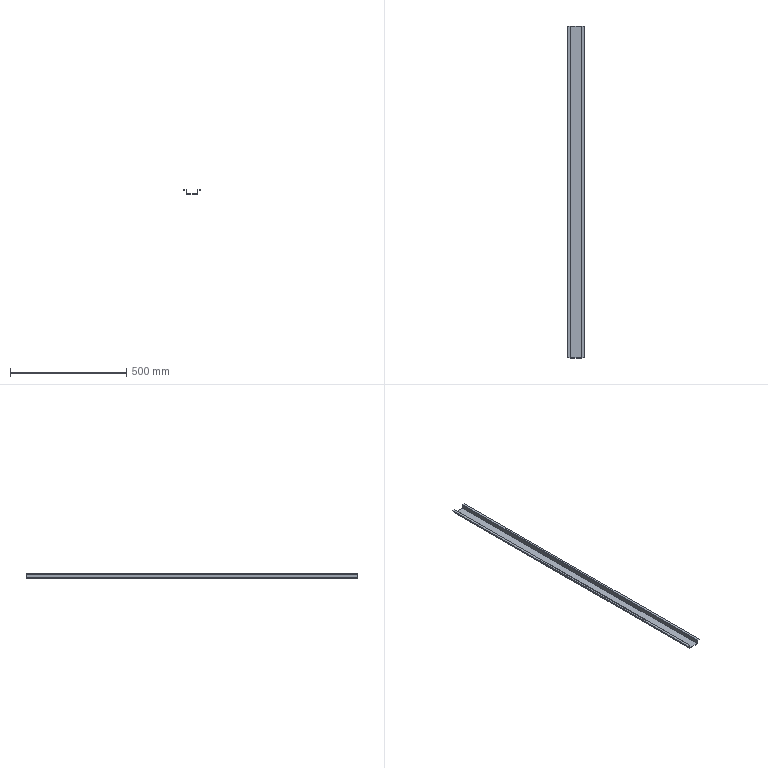Component | SolidWorks | AirFurnaceElectricalCabinet-ElectricalPanelAssembly-1_ElectricalPanelReinforcementPlate-L1425-1 | 1 solid | 38 faces | box 71.6 x 1425 x 18 mm | volume 175929 mm3 | plane 30 | cylinder 8 | commonest cylinder face diameters 3.9 x4 1.5 x4
STEP:
#1=CARTESIAN_POINT('',(8.781,4.854,-4.843));
#2=VERTEX_POINT('',#1);
#3=CARTESIAN_POINT('',(6.967,4.854,-4.843));
#4=VERTEX_POINT('',#3);
#5=CARTESIAN_POINT('',(8.858,4.854,-4.843));
#6=DIRECTION('',(-1.,0.,0.));
#7=VECTOR('',#6,39.37);
#8=LINE('',#5,#7);
#9=EDGE_CURVE('',#2,#4,#8,.T.);
#10=ORIENTED_EDGE('',*,*,#9,.F.);
#11=CARTESIAN_POINT('',(8.781,4.854,-4.795));
#12=VERTEX_POINT('',#11);
#13=CARTESIAN_POINT('',(8.781,4.854,-4.843));
#14=DIRECTION('',(0.,0.,1.));
#15=VECTOR('',#14,39.37);
#16=LINE('',#13,#15);
#17=EDGE_CURVE('',#2,#12,#16,.T.);
#18=ORIENTED_EDGE('',*,*,#17,.T.);
#19=CARTESIAN_POINT('',(6.967,4.854,-4.795));
#20=VERTEX_POINT('',#19);
#21=CARTESIAN_POINT('',(8.858,4.854,-4.795));
#22=DIRECTION('',(-1.,0.,0.));
#23=VECTOR('',#22,39.37);
#24=LINE('',#21,#23);
#25=EDGE_CURVE('',#12,#20,#24,.T.);
#26=ORIENTED_EDGE('',*,*,#25,.T.);
#27=CARTESIAN_POINT('',(6.967,4.854,-4.795));
#28=DIRECTION('',(-0.,0.,-1.));
#29=VECTOR('',#28,39.37);
#30=LINE('',#27,#29);
#31=EDGE_CURVE('',#20,#4,#30,.T.);
#32=ORIENTED_EDGE('',*,*,#31,.T.);
#33=EDGE_LOOP('',(#10,#18,#26,#32));
#34=FACE_OUTER_BOUND('',#33,.T.);
#35=CARTESIAN_POINT('',(8.811,4.854,-4.766));
#36=DIRECTION('',(0.,-1.,0.));
#37=DIRECTION('',(-1.,0.,0.));
#38=AXIS2_PLACEMENT_3D('',#35,#36,#37);
#39=PLANE('',#38);
#40=ADVANCED_FACE('',(#34),#39,.T.);
#41=CARTESIAN_POINT('',(8.781,60.957,-4.843));
#42=VERTEX_POINT('',#41);
#43=CARTESIAN_POINT('',(6.967,60.957,-4.843));
#44=VERTEX_POINT('',#43);
#45=CARTESIAN_POINT('',(8.858,60.957,-4.843));
#46=DIRECTION('',(-1.,0.,0.));
#47=VECTOR('',#46,39.37);
#48=LINE('',#45,#47);
#49=EDGE_CURVE('',#42,#44,#48,.T.);
#50=ORIENTED_EDGE('',*,*,#49,.T.);
#51=CARTESIAN_POINT('',(6.967,60.957,-4.795));
#52=VERTEX_POINT('',#51);
#53=CARTESIAN_POINT('',(6.967,60.957,-4.843));
#54=DIRECTION('',(0.,0.,1.));
#55=VECTOR('',#54,39.37);
#56=LINE('',#53,#55);
#57=EDGE_CURVE('',#44,#52,#56,.T.);
#58=ORIENTED_EDGE('',*,*,#57,.T.);
#59=CARTESIAN_POINT('',(8.781,60.957,-4.795));
#60=VERTEX_POINT('',#59);
#61=CARTESIAN_POINT('',(8.858,60.957,-4.795));
#62=DIRECTION('',(-1.,0.,0.));
#63=VECTOR('',#62,39.37);
#64=LINE('',#61,#63);
#65=EDGE_CURVE('',#60,#52,#64,.T.);
#66=ORIENTED_EDGE('',*,*,#65,.F.);
#67=CARTESIAN_POINT('',(8.781,60.957,-4.795));
#68=DIRECTION('',(-0.,0.,-1.));
#69=VECTOR('',#68,39.37);
#70=LINE('',#67,#69);
#71=EDGE_CURVE('',#60,#42,#70,.T.);
#72=ORIENTED_EDGE('',*,*,#71,.T.);
#73=EDGE_LOOP('',(#50,#58,#66,#72));
#74=FACE_OUTER_BOUND('',#73,.T.);
#75=CARTESIAN_POINT('',(6.937,60.957,-4.766));
#76=DIRECTION('',(0.,1.,0.));
#77=DIRECTION('',(1.,0.,-0.));
#78=AXIS2_PLACEMENT_3D('',#75,#76,#77);
#79=PLANE('',#78);
#80=ADVANCED_FACE('',(#74),#79,.T.);
#81=ORIENTED_EDGE('',*,*,#49,.F.);
#82=CARTESIAN_POINT('',(8.781,4.854,-4.843));
#83=DIRECTION('',(0.,1.,0.));
#84=VECTOR('',#83,39.37);
#85=LINE('',#82,#84);
#86=EDGE_CURVE('',#2,#42,#85,.T.);
#87=ORIENTED_EDGE('',*,*,#86,.F.);
#88=ORIENTED_EDGE('',*,*,#9,.T.);
#89=CARTESIAN_POINT('',(6.967,4.854,-4.843));
#90=DIRECTION('',(0.,1.,0.));
#91=VECTOR('',#90,39.37);
#92=LINE('',#89,#91);
#93=EDGE_CURVE('',#4,#44,#92,.T.);
#94=ORIENTED_EDGE('',*,*,#93,.T.);
#95=EDGE_LOOP('',(#81,#87,#88,#94));
#96=FACE_OUTER_BOUND('',#95,.T.);
#97=CARTESIAN_POINT('',(8.858,4.854,-4.843));
#98=DIRECTION('',(-0.,0.,-1.));
#99=DIRECTION('',(1.,0.,-0.));
#100=AXIS2_PLACEMENT_3D('',#97,#98,#99);
#101=PLANE('',#100);
#102=ADVANCED_FACE('',(#96),#101,.T.);
#103=ORIENTED_EDGE('',*,*,#65,.T.);
#104=CARTESIAN_POINT('',(6.967,4.854,-4.795));
#105=DIRECTION('',(0.,1.,0.));
#106=VECTOR('',#105,39.37);
#107=LINE('',#104,#106);
#108=EDGE_CURVE('',#20,#52,#107,.T.);
#109=ORIENTED_EDGE('',*,*,#108,.F.);
#110=ORIENTED_EDGE('',*,*,#25,.F.);
#111=CARTESIAN_POINT('',(8.781,4.854,-4.795));
#112=DIRECTION('',(0.,1.,0.));
#113=VECTOR('',#112,39.37);
#114=LINE('',#111,#113);
#115=EDGE_CURVE('',#12,#60,#114,.T.);
#116=ORIENTED_EDGE('',*,*,#115,.T.);
#117=EDGE_LOOP('',(#103,#109,#110,#116));
#118=FACE_OUTER_BOUND('',#117,.T.);
#119=CARTESIAN_POINT('',(8.858,4.854,-4.795));
#120=DIRECTION('',(-0.,0.,-1.));
#121=DIRECTION('',(1.,0.,-0.));
#122=AXIS2_PLACEMENT_3D('',#119,#120,#121);
#123=PLANE('',#122);
#124=ADVANCED_FACE('',(#118),#123,.F.);
#125=ORIENTED_EDGE('',*,*,#31,.F.);
#126=CARTESIAN_POINT('',(6.937,4.854,-4.766));
#127=VERTEX_POINT('',#126);
#128=CARTESIAN_POINT('',(6.967,4.854,-4.766));
#129=DIRECTION('',(0.,1.,0.));
#130=DIRECTION('',(1.,0.,0.));
#131=AXIS2_PLACEMENT_3D('',#128,#129,#130);
#132=CIRCLE('',#131,0.02953);
#133=EDGE_CURVE('',#20,#127,#132,.T.);
#134=ORIENTED_EDGE('',*,*,#133,.T.);
#135=CARTESIAN_POINT('',(6.89,4.854,-4.766));
#136=VERTEX_POINT('',#135);
#137=CARTESIAN_POINT('',(6.89,4.854,-4.766));
#138=DIRECTION('',(1.,0.,-0.));
#139=VECTOR('',#138,39.37);
#140=LINE('',#137,#139);
#141=EDGE_CURVE('',#136,#127,#140,.T.);
#142=ORIENTED_EDGE('',*,*,#141,.F.);
#143=CARTESIAN_POINT('',(6.967,4.854,-4.766));
#144=DIRECTION('',(0.,1.,0.));
#145=DIRECTION('',(1.,0.,0.));
#146=AXIS2_PLACEMENT_3D('',#143,#144,#145);
#147=CIRCLE('',#146,0.07677);
#148=EDGE_CURVE('',#4,#136,#147,.T.);
#149=ORIENTED_EDGE('',*,*,#148,.F.);
#150=EDGE_LOOP('',(#125,#134,#142,#149));
#151=FACE_OUTER_BOUND('',#150,.T.);
#152=CARTESIAN_POINT('',(6.967,4.854,-4.766));
#153=DIRECTION('',(0.,-1.,0.));
#154=DIRECTION('',(-1.,0.,0.));
#155=AXIS2_PLACEMENT_3D('',#152,#153,#154);
#156=PLANE('',#155);
#157=ADVANCED_FACE('',(#151),#156,.T.);
#158=CARTESIAN_POINT('',(6.937,60.957,-4.766));
#159=VERTEX_POINT('',#158);
#160=CARTESIAN_POINT('',(6.89,60.957,-4.766));
#161=VERTEX_POINT('',#160);
#162=CARTESIAN_POINT('',(6.937,60.957,-4.766));
#163=DIRECTION('',(-1.,0.,0.));
#164=VECTOR('',#163,39.37);
#165=LINE('',#162,#164);
#166=EDGE_CURVE('',#159,#161,#165,.T.);
#167=ORIENTED_EDGE('',*,*,#166,.F.);
#168=CARTESIAN_POINT('',(6.967,60.957,-4.766));
#169=DIRECTION('',(0.,-1.,0.));
#170=DIRECTION('',(1.,0.,0.));
#171=AXIS2_PLACEMENT_3D('',#168,#169,#170);
#172=CIRCLE('',#171,0.02953);
#173=EDGE_CURVE('',#159,#52,#172,.T.);
#174=ORIENTED_EDGE('',*,*,#173,.T.);
#175=ORIENTED_EDGE('',*,*,#57,.F.);
#176=CARTESIAN_POINT('',(6.967,60.957,-4.766));
#177=DIRECTION('',(0.,-1.,0.));
#178=DIRECTION('',(-1.,0.,0.));
#179=AXIS2_PLACEMENT_3D('',#176,#177,#178);
#180=CIRCLE('',#179,0.07677);
#181=EDGE_CURVE('',#161,#44,#180,.T.);
#182=ORIENTED_EDGE('',*,*,#181,.F.);
#183=EDGE_LOOP('',(#167,#174,#175,#182));
#184=FACE_OUTER_BOUND('',#183,.T.);
#185=CARTESIAN_POINT('',(6.967,60.957,-4.766));
#186=DIRECTION('',(0.,1.,0.));
#187=DIRECTION('',(1.,0.,-0.));
#188=AXIS2_PLACEMENT_3D('',#185,#186,#187);
#189=PLANE('',#188);
#190=ADVANCED_FACE('',(#184),#189,.T.);
#191=ORIENTED_EDGE('',*,*,#181,.T.);
#192=ORIENTED_EDGE('',*,*,#93,.F.);
#193=ORIENTED_EDGE('',*,*,#148,.T.);
#194=CARTESIAN_POINT('',(6.89,4.854,-4.766));
#195=DIRECTION('',(0.,1.,0.));
#196=VECTOR('',#195,39.37);
#197=LINE('',#194,#196);
#198=EDGE_CURVE('',#136,#161,#197,.T.);
#199=ORIENTED_EDGE('',*,*,#198,.T.);
#200=EDGE_LOOP('',(#191,#192,#193,#199));
#201=FACE_OUTER_BOUND('',#200,.T.);
#202=CARTESIAN_POINT('',(6.967,-23.197,-4.766));
#203=DIRECTION('',(0.,1.,0.));
#204=DIRECTION('',(1.,0.,0.));
#205=AXIS2_PLACEMENT_3D('',#202,#203,#204);
#206=CYLINDRICAL_SURFACE('',#205,0.07677);
#207=ADVANCED_FACE('',(#201),#206,.T.);
#208=ORIENTED_EDGE('',*,*,#173,.F.);
#209=CARTESIAN_POINT('',(6.937,4.854,-4.766));
#210=DIRECTION('',(0.,1.,0.));
#211=VECTOR('',#210,39.37);
#212=LINE('',#209,#211);
#213=EDGE_CURVE('',#127,#159,#212,.T.);
#214=ORIENTED_EDGE('',*,*,#213,.F.);
#215=ORIENTED_EDGE('',*,*,#133,.F.);
#216=ORIENTED_EDGE('',*,*,#108,.T.);
#217=EDGE_LOOP('',(#208,#214,#215,#216));
#218=FACE_OUTER_BOUND('',#217,.T.);
#219=CARTESIAN_POINT('',(6.967,-23.197,-4.766));
#220=DIRECTION('',(0.,1.,0.));
#221=DIRECTION('',(1.,0.,0.));
#222=AXIS2_PLACEMENT_3D('',#219,#220,#221);
#223=CYLINDRICAL_SURFACE('',#222,0.02953);
#224=ADVANCED_FACE('',(#218),#223,.F.);
#225=CARTESIAN_POINT('',(6.465,60.957,-4.181));
#226=VERTEX_POINT('',#225);
#227=CARTESIAN_POINT('',(6.465,60.957,-4.134));
#228=VERTEX_POINT('',#227);
#229=CARTESIAN_POINT('',(6.465,60.957,-4.181));
#230=DIRECTION('',(0.,0.,1.));
#231=VECTOR('',#230,39.37);
#232=LINE('',#229,#231);
#233=EDGE_CURVE('',#226,#228,#232,.T.);
#234=ORIENTED_EDGE('',*,*,#233,.F.);
#235=CARTESIAN_POINT('',(6.465,4.854,-4.181));
#236=VERTEX_POINT('',#235);
#237=CARTESIAN_POINT('',(6.465,4.854,-4.181));
#238=DIRECTION('',(0.,1.,0.));
#239=VECTOR('',#238,39.37);
#240=LINE('',#237,#239);
#241=EDGE_CURVE('',#236,#226,#240,.T.);
#242=ORIENTED_EDGE('',*,*,#241,.F.);
#243=CARTESIAN_POINT('',(6.465,4.854,-4.134));
#244=VERTEX_POINT('',#243);
#245=CARTESIAN_POINT('',(6.465,4.854,-4.181));
#246=DIRECTION('',(0.,0.,1.));
#247=VECTOR('',#246,39.37);
#248=LINE('',#245,#247);
#249=EDGE_CURVE('',#236,#244,#248,.T.);
#250=ORIENTED_EDGE('',*,*,#249,.T.);
#251=CARTESIAN_POINT('',(6.465,4.854,-4.134));
#252=DIRECTION('',(0.,1.,0.));
#253=VECTOR('',#252,39.37);
#254=LINE('',#251,#253);
#255=EDGE_CURVE('',#244,#228,#254,.T.);
#256=ORIENTED_EDGE('',*,*,#255,.T.);
#257=EDGE_LOOP('',(#234,#242,#250,#256));
#258=FACE_OUTER_BOUND('',#257,.T.);
#259=CARTESIAN_POINT('',(6.465,4.854,-4.181));
#260=DIRECTION('',(-1.,0.,0.));
#261=DIRECTION('',(0.,1.,0.));
#262=AXIS2_PLACEMENT_3D('',#259,#260,#261);
#263=PLANE('',#262);
#264=ADVANCED_FACE('',(#258),#263,.T.);
#265=CARTESIAN_POINT('',(6.86,60.957,-4.134));
#266=VERTEX_POINT('',#265);
#267=CARTESIAN_POINT('',(6.89,60.957,-4.134));
#268=DIRECTION('',(-1.,0.,0.));
#269=VECTOR('',#268,39.37);
#270=LINE('',#267,#269);
#271=EDGE_CURVE('',#266,#228,#270,.T.);
#272=ORIENTED_EDGE('',*,*,#271,.F.);
#273=CARTESIAN_POINT('',(6.86,60.957,-4.181));
#274=VERTEX_POINT('',#273);
#275=CARTESIAN_POINT('',(6.86,60.957,-4.134));
#276=DIRECTION('',(-0.,0.,-1.));
#277=VECTOR('',#276,39.37);
#278=LINE('',#275,#277);
#279=EDGE_CURVE('',#266,#274,#278,.T.);
#280=ORIENTED_EDGE('',*,*,#279,.T.);
#281=CARTESIAN_POINT('',(6.89,60.957,-4.181));
#282=DIRECTION('',(-1.,0.,0.));
#283=VECTOR('',#282,39.37);
#284=LINE('',#281,#283);
#285=EDGE_CURVE('',#274,#226,#284,.T.);
#286=ORIENTED_EDGE('',*,*,#285,.T.);
#287=ORIENTED_EDGE('',*,*,#233,.T.);
#288=EDGE_LOOP('',(#272,#280,#286,#287));
#289=FACE_OUTER_BOUND('',#288,.T.);
#290=CARTESIAN_POINT('',(6.86,60.957,-4.211));
#291=DIRECTION('',(0.,1.,0.));
#292=DIRECTION('',(1.,0.,-0.));
#293=AXIS2_PLACEMENT_3D('',#290,#291,#292);
#294=PLANE('',#293);
#295=ADVANCED_FACE('',(#289),#294,.T.);
#296=ORIENTED_EDGE('',*,*,#271,.T.);
#297=ORIENTED_EDGE('',*,*,#255,.F.);
#298=CARTESIAN_POINT('',(6.86,4.854,-4.134));
#299=VERTEX_POINT('',#298);
#300=CARTESIAN_POINT('',(6.89,4.854,-4.134));
#301=DIRECTION('',(-1.,0.,0.));
#302=VECTOR('',#301,39.37);
#303=LINE('',#300,#302);
#304=EDGE_CURVE('',#299,#244,#303,.T.);
#305=ORIENTED_EDGE('',*,*,#304,.F.);
#306=CARTESIAN_POINT('',(6.86,4.854,-4.134));
#307=DIRECTION('',(0.,1.,0.));
#308=VECTOR('',#307,39.37);
#309=LINE('',#306,#308);
#310=EDGE_CURVE('',#299,#266,#309,.T.);
#311=ORIENTED_EDGE('',*,*,#310,.T.);
#312=EDGE_LOOP('',(#296,#297,#305,#311));
#313=FACE_OUTER_BOUND('',#312,.T.);
#314=CARTESIAN_POINT('',(6.89,4.854,-4.134));
#315=DIRECTION('',(0.,0.,-1.));
#316=DIRECTION('',(1.,0.,0.));
#317=AXIS2_PLACEMENT_3D('',#314,#315,#316);
#318=PLANE('',#317);
#319=ADVANCED_FACE('',(#313),#318,.F.);
#320=CARTESIAN_POINT('',(6.86,4.854,-4.181));
#321=VERTEX_POINT('',#320);
#322=CARTESIAN_POINT('',(6.89,4.854,-4.181));
#323=DIRECTION('',(-1.,0.,0.));
#324=VECTOR('',#323,39.37);
#325=LINE('',#322,#324);
#326=EDGE_CURVE('',#321,#236,#325,.T.);
#327=ORIENTED_EDGE('',*,*,#326,.F.);
#328=CARTESIAN_POINT('',(6.86,4.854,-4.181));
#329=DIRECTION('',(0.,0.,1.));
#330=VECTOR('',#329,39.37);
#331=LINE('',#328,#330);
#332=EDGE_CURVE('',#321,#299,#331,.T.);
#333=ORIENTED_EDGE('',*,*,#332,.T.);
#334=ORIENTED_EDGE('',*,*,#304,.T.);
#335=ORIENTED_EDGE('',*,*,#249,.F.);
#336=EDGE_LOOP('',(#327,#333,#334,#335));
#337=FACE_OUTER_BOUND('',#336,.T.);
#338=CARTESIAN_POINT('',(6.937,4.854,-4.211));
#339=DIRECTION('',(0.,-1.,0.));
#340=DIRECTION('',(-1.,0.,0.));
#341=AXIS2_PLACEMENT_3D('',#338,#339,#340);
#342=PLANE('',#341);
#343=ADVANCED_FACE('',(#337),#342,.T.);
#344=ORIENTED_EDGE('',*,*,#285,.F.);
#345=CARTESIAN_POINT('',(6.86,4.854,-4.181));
#346=DIRECTION('',(0.,1.,0.));
#347=VECTOR('',#346,39.37);
#348=LINE('',#345,#347);
#349=EDGE_CURVE('',#321,#274,#348,.T.);
#350=ORIENTED_EDGE('',*,*,#349,.F.);
#351=ORIENTED_EDGE('',*,*,#326,.T.);
#352=ORIENTED_EDGE('',*,*,#241,.T.);
#353=EDGE_LOOP('',(#344,#350,#351,#352));
#354=FACE_OUTER_BOUND('',#353,.T.);
#355=CARTESIAN_POINT('',(6.89,4.854,-4.181));
#356=DIRECTION('',(0.,0.,-1.));
#357=DIRECTION('',(1.,0.,0.));
#358=AXIS2_PLACEMENT_3D('',#355,#356,#357);
#359=PLANE('',#358);
#360=ADVANCED_FACE('',(#354),#359,.T.);
#361=ORIENTED_EDGE('',*,*,#279,.F.);
#362=CARTESIAN_POINT('',(6.937,60.957,-4.211));
#363=VERTEX_POINT('',#362);
#364=CARTESIAN_POINT('',(6.86,60.957,-4.211));
#365=DIRECTION('',(0.,1.,0.));
#366=DIRECTION('',(0.,0.,-1.));
#367=AXIS2_PLACEMENT_3D('',#364,#365,#366);
#368=CIRCLE('',#367,0.07677);
#369=EDGE_CURVE('',#266,#363,#368,.T.);
#370=ORIENTED_EDGE('',*,*,#369,.T.);
#371=CARTESIAN_POINT('',(6.89,60.957,-4.211));
#372=VERTEX_POINT('',#371);
#373=CARTESIAN_POINT('',(6.89,60.957,-4.211));
#374=DIRECTION('',(1.,0.,-0.));
#375=VECTOR('',#374,39.37);
#376=LINE('',#373,#375);
#377=EDGE_CURVE('',#372,#363,#376,.T.);
#378=ORIENTED_EDGE('',*,*,#377,.F.);
#379=CARTESIAN_POINT('',(6.86,60.957,-4.211));
#380=DIRECTION('',(0.,1.,0.));
#381=DIRECTION('',(0.,0.,-1.));
#382=AXIS2_PLACEMENT_3D('',#379,#380,#381);
#383=CIRCLE('',#382,0.02953);
#384=EDGE_CURVE('',#274,#372,#383,.T.);
#385=ORIENTED_EDGE('',*,*,#384,.F.);
#386=EDGE_LOOP('',(#361,#370,#378,#385));
#387=FACE_OUTER_BOUND('',#386,.T.);
#388=CARTESIAN_POINT('',(6.86,60.957,-4.211));
#389=DIRECTION('',(0.,-1.,0.));
#390=DIRECTION('',(-0.,0.,1.));
#391=AXIS2_PLACEMENT_3D('',#388,#389,#390);
#392=PLANE('',#391);
#393=ADVANCED_FACE('',(#387),#392,.F.);
#394=ORIENTED_EDGE('',*,*,#369,.F.);
#395=ORIENTED_EDGE('',*,*,#310,.F.);
#396=CARTESIAN_POINT('',(6.937,4.854,-4.211));
#397=VERTEX_POINT('',#396);
#398=CARTESIAN_POINT('',(6.86,4.854,-4.211));
#399=DIRECTION('',(0.,-1.,0.));
#400=DIRECTION('',(0.,0.,-1.));
#401=AXIS2_PLACEMENT_3D('',#398,#399,#400);
#402=CIRCLE('',#401,0.07677);
#403=EDGE_CURVE('',#397,#299,#402,.T.);
#404=ORIENTED_EDGE('',*,*,#403,.F.);
#405=CARTESIAN_POINT('',(6.937,4.854,-4.211));
#406=DIRECTION('',(0.,1.,0.));
#407=VECTOR('',#406,39.37);
#408=LINE('',#405,#407);
#409=EDGE_CURVE('',#397,#363,#408,.T.);
#410=ORIENTED_EDGE('',*,*,#409,.T.);
#411=EDGE_LOOP('',(#394,#395,#404,#410));
#412=FACE_OUTER_BOUND('',#411,.T.);
#413=CARTESIAN_POINT('',(6.86,-23.197,-4.211));
#414=DIRECTION('',(0.,1.,0.));
#415=DIRECTION('',(0.,0.,-1.));
#416=AXIS2_PLACEMENT_3D('',#413,#414,#415);
#417=CYLINDRICAL_SURFACE('',#416,0.07677);
#418=ADVANCED_FACE('',(#412),#417,.T.);
#419=CARTESIAN_POINT('',(6.89,4.854,-4.211));
#420=VERTEX_POINT('',#419);
#421=CARTESIAN_POINT('',(6.937,4.854,-4.211));
#422=DIRECTION('',(-1.,0.,0.));
#423=VECTOR('',#422,39.37);
#424=LINE('',#421,#423);
#425=EDGE_CURVE('',#397,#420,#424,.T.);
#426=ORIENTED_EDGE('',*,*,#425,.F.);
#427=ORIENTED_EDGE('',*,*,#403,.T.);
#428=ORIENTED_EDGE('',*,*,#332,.F.);
#429=CARTESIAN_POINT('',(6.86,4.854,-4.211));
#430=DIRECTION('',(0.,-1.,0.));
#431=DIRECTION('',(0.,0.,1.));
#432=AXIS2_PLACEMENT_3D('',#429,#430,#431);
#433=CIRCLE('',#432,0.02953);
#434=EDGE_CURVE('',#420,#321,#433,.T.);
#435=ORIENTED_EDGE('',*,*,#434,.F.);
#436=EDGE_LOOP('',(#426,#427,#428,#435));
#437=FACE_OUTER_BOUND('',#436,.T.);
#438=CARTESIAN_POINT('',(6.86,4.854,-4.211));
#439=DIRECTION('',(0.,1.,0.));
#440=DIRECTION('',(0.,0.,-1.));
#441=AXIS2_PLACEMENT_3D('',#438,#439,#440);
#442=PLANE('',#441);
#443=ADVANCED_FACE('',(#437),#442,.F.);
#444=ORIENTED_EDGE('',*,*,#384,.T.);
#445=CARTESIAN_POINT('',(6.89,4.854,-4.211));
#446=DIRECTION('',(0.,1.,0.));
#447=VECTOR('',#446,39.37);
#448=LINE('',#445,#447);
#449=EDGE_CURVE('',#420,#372,#448,.T.);
#450=ORIENTED_EDGE('',*,*,#449,.F.);
#451=ORIENTED_EDGE('',*,*,#434,.T.);
#452=ORIENTED_EDGE('',*,*,#349,.T.);
#453=EDGE_LOOP('',(#444,#450,#451,#452));
#454=FACE_OUTER_BOUND('',#453,.T.);
#455=CARTESIAN_POINT('',(6.86,-23.197,-4.211));
#456=DIRECTION('',(0.,1.,0.));
#457=DIRECTION('',(0.,0.,-1.));
#458=AXIS2_PLACEMENT_3D('',#455,#456,#457);
#459=CYLINDRICAL_SURFACE('',#458,0.02953);
#460=ADVANCED_FACE('',(#454),#459,.F.);
#461=CARTESIAN_POINT('',(6.89,60.957,-4.843));
#462=DIRECTION('',(0.,0.,1.));
#463=VECTOR('',#462,39.37);
#464=LINE('',#461,#463);
#465=EDGE_CURVE('',#161,#372,#464,.T.);
#466=ORIENTED_EDGE('',*,*,#465,.F.);
#467=ORIENTED_EDGE('',*,*,#198,.F.);
#468=CARTESIAN_POINT('',(6.89,4.854,-4.843));
#469=DIRECTION('',(0.,0.,1.));
#470=VECTOR('',#469,39.37);
#471=LINE('',#468,#470);
#472=EDGE_CURVE('',#136,#420,#471,.T.);
#473=ORIENTED_EDGE('',*,*,#472,.T.);
#474=ORIENTED_EDGE('',*,*,#449,.T.);
#475=EDGE_LOOP('',(#466,#467,#473,#474));
#476=FACE_OUTER_BOUND('',#475,.T.);
#477=CARTESIAN_POINT('',(6.89,4.854,-4.843));
#478=DIRECTION('',(-1.,0.,0.));
#479=DIRECTION('',(0.,1.,0.));
#480=AXIS2_PLACEMENT_3D('',#477,#478,#479);
#481=PLANE('',#480);
#482=ADVANCED_FACE('',(#476),#481,.T.);
#483=ORIENTED_EDGE('',*,*,#472,.F.);
#484=ORIENTED_EDGE('',*,*,#141,.T.);
#485=CARTESIAN_POINT('',(6.937,4.854,-4.843));
#486=DIRECTION('',(0.,0.,1.));
#487=VECTOR('',#486,39.37);
#488=LINE('',#485,#487);
#489=EDGE_CURVE('',#127,#397,#488,.T.);
#490=ORIENTED_EDGE('',*,*,#489,.T.);
#491=ORIENTED_EDGE('',*,*,#425,.T.);
#492=EDGE_LOOP('',(#483,#484,#490,#491));
#493=FACE_OUTER_BOUND('',#492,.T.);
#494=CARTESIAN_POINT('',(6.967,4.854,-4.795));
#495=DIRECTION('',(0.,-1.,0.));
#496=DIRECTION('',(-1.,0.,0.));
#497=AXIS2_PLACEMENT_3D('',#494,#495,#496);
#498=PLANE('',#497);
#499=ADVANCED_FACE('',(#493),#498,.T.);
#500=CARTESIAN_POINT('',(6.937,60.957,-4.843));
#501=DIRECTION('',(0.,0.,1.));
#502=VECTOR('',#501,39.37);
#503=LINE('',#500,#502);
#504=EDGE_CURVE('',#159,#363,#503,.T.);
#505=ORIENTED_EDGE('',*,*,#504,.T.);
#506=ORIENTED_EDGE('',*,*,#409,.F.);
#507=ORIENTED_EDGE('',*,*,#489,.F.);
#508=ORIENTED_EDGE('',*,*,#213,.T.);
#509=EDGE_LOOP('',(#505,#506,#507,#508));
#510=FACE_OUTER_BOUND('',#509,.T.);
#511=CARTESIAN_POINT('',(6.937,4.854,-4.843));
#512=DIRECTION('',(-1.,0.,0.));
#513=DIRECTION('',(0.,1.,0.));
#514=AXIS2_PLACEMENT_3D('',#511,#512,#513);
#515=PLANE('',#514);
#516=ADVANCED_FACE('',(#510),#515,.F.);
#517=ORIENTED_EDGE('',*,*,#465,.T.);
#518=ORIENTED_EDGE('',*,*,#377,.T.);
#519=ORIENTED_EDGE('',*,*,#504,.F.);
#520=ORIENTED_EDGE('',*,*,#166,.T.);
#521=EDGE_LOOP('',(#517,#518,#519,#520));
#522=FACE_OUTER_BOUND('',#521,.T.);
#523=CARTESIAN_POINT('',(6.86,60.957,-4.134));
#524=DIRECTION('',(0.,1.,0.));
#525=DIRECTION('',(1.,0.,-0.));
#526=AXIS2_PLACEMENT_3D('',#523,#524,#525);
#527=PLANE('',#526);
#528=ADVANCED_FACE('',(#522),#527,.T.);
#529=CARTESIAN_POINT('',(8.811,4.854,-4.766));
#530=VERTEX_POINT('',#529);
#531=CARTESIAN_POINT('',(8.858,4.854,-4.766));
#532=VERTEX_POINT('',#531);
#533=CARTESIAN_POINT('',(8.811,4.854,-4.766));
#534=DIRECTION('',(1.,0.,-0.));
#535=VECTOR('',#534,39.37);
#536=LINE('',#533,#535);
#537=EDGE_CURVE('',#530,#532,#536,.T.);
#538=ORIENTED_EDGE('',*,*,#537,.F.);
#539=CARTESIAN_POINT('',(8.781,4.854,-4.766));
#540=DIRECTION('',(0.,1.,0.));
#541=DIRECTION('',(-1.,0.,0.));
#542=AXIS2_PLACEMENT_3D('',#539,#540,#541);
#543=CIRCLE('',#542,0.02953);
#544=EDGE_CURVE('',#530,#12,#543,.T.);
#545=ORIENTED_EDGE('',*,*,#544,.T.);
#546=ORIENTED_EDGE('',*,*,#17,.F.);
#547=CARTESIAN_POINT('',(8.781,4.854,-4.766));
#548=DIRECTION('',(0.,1.,0.));
#549=DIRECTION('',(1.,0.,0.));
#550=AXIS2_PLACEMENT_3D('',#547,#548,#549);
#551=CIRCLE('',#550,0.07677);
#552=EDGE_CURVE('',#532,#2,#551,.T.);
#553=ORIENTED_EDGE('',*,*,#552,.F.);
#554=EDGE_LOOP('',(#538,#545,#546,#553));
#555=FACE_OUTER_BOUND('',#554,.T.);
#556=CARTESIAN_POINT('',(8.781,4.854,-4.766));
#557=DIRECTION('',(0.,-1.,0.));
#558=DIRECTION('',(-1.,0.,0.));
#559=AXIS2_PLACEMENT_3D('',#556,#557,#558);
#560=PLANE('',#559);
#561=ADVANCED_FACE('',(#555),#560,.T.);
#562=ORIENTED_EDGE('',*,*,#71,.F.);
#563=CARTESIAN_POINT('',(8.811,60.957,-4.766));
#564=VERTEX_POINT('',#563);
#565=CARTESIAN_POINT('',(8.781,60.957,-4.766));
#566=DIRECTION('',(0.,-1.,0.));
#567=DIRECTION('',(-1.,0.,0.));
#568=AXIS2_PLACEMENT_3D('',#565,#566,#567);
#569=CIRCLE('',#568,0.02953);
#570=EDGE_CURVE('',#60,#564,#569,.T.);
#571=ORIENTED_EDGE('',*,*,#570,.T.);
#572=CARTESIAN_POINT('',(8.858,60.957,-4.766));
#573=VERTEX_POINT('',#572);
#574=CARTESIAN_POINT('',(8.858,60.957,-4.766));
#575=DIRECTION('',(-1.,0.,0.));
#576=VECTOR('',#575,39.37);
#577=LINE('',#574,#576);
#578=EDGE_CURVE('',#573,#564,#577,.T.);
#579=ORIENTED_EDGE('',*,*,#578,.F.);
#580=CARTESIAN_POINT('',(8.781,60.957,-4.766));
#581=DIRECTION('',(0.,-1.,0.));
#582=DIRECTION('',(-1.,0.,0.));
#583=AXIS2_PLACEMENT_3D('',#580,#581,#582);
#584=CIRCLE('',#583,0.07677);
#585=EDGE_CURVE('',#42,#573,#584,.T.);
#586=ORIENTED_EDGE('',*,*,#585,.F.);
#587=EDGE_LOOP('',(#562,#571,#579,#586));
#588=FACE_OUTER_BOUND('',#587,.T.);
#589=CARTESIAN_POINT('',(8.781,60.957,-4.766));
#590=DIRECTION('',(0.,1.,0.));
#591=DIRECTION('',(1.,0.,-0.));
#592=AXIS2_PLACEMENT_3D('',#589,#590,#591);
#593=PLANE('',#592);
#594=ADVANCED_FACE('',(#588),#593,.T.);
#595=ORIENTED_EDGE('',*,*,#585,.T.);
#596=CARTESIAN_POINT('',(8.858,4.854,-4.766));
#597=DIRECTION('',(0.,1.,0.));
#598=VECTOR('',#597,39.37);
#599=LINE('',#596,#598);
#600=EDGE_CURVE('',#532,#573,#599,.T.);
#601=ORIENTED_EDGE('',*,*,#600,.F.);
#602=ORIENTED_EDGE('',*,*,#552,.T.);
#603=ORIENTED_EDGE('',*,*,#86,.T.);
#604=EDGE_LOOP('',(#595,#601,#602,#603));
#605=FACE_OUTER_BOUND('',#604,.T.);
#606=CARTESIAN_POINT('',(8.781,89.008,-4.766));
#607=DIRECTION('',(0.,-1.,0.));
#608=DIRECTION('',(-1.,0.,0.));
#609=AXIS2_PLACEMENT_3D('',#606,#607,#608);
#610=CYLINDRICAL_SURFACE('',#609,0.07677);
#611=ADVANCED_FACE('',(#605),#610,.T.);
#612=ORIENTED_EDGE('',*,*,#570,.F.);
#613=ORIENTED_EDGE('',*,*,#115,.F.);
#614=ORIENTED_EDGE('',*,*,#544,.F.);
#615=CARTESIAN_POINT('',(8.811,4.854,-4.766));
#616=DIRECTION('',(0.,1.,0.));
#617=VECTOR('',#616,39.37);
#618=LINE('',#615,#617);
#619=EDGE_CURVE('',#530,#564,#618,.T.);
#620=ORIENTED_EDGE('',*,*,#619,.T.);
#621=EDGE_LOOP('',(#612,#613,#614,#620));
#622=FACE_OUTER_BOUND('',#621,.T.);
#623=CARTESIAN_POINT('',(8.781,89.008,-4.766));
#624=DIRECTION('',(0.,-1.,0.));
#625=DIRECTION('',(-1.,0.,0.));
#626=AXIS2_PLACEMENT_3D('',#623,#624,#625);
#627=CYLINDRICAL_SURFACE('',#626,0.02953);
#628=ADVANCED_FACE('',(#622),#627,.F.);
#629=CARTESIAN_POINT('',(8.858,60.957,-4.211));
#630=VERTEX_POINT('',#629);
#631=CARTESIAN_POINT('',(8.858,60.957,-4.181));
#632=DIRECTION('',(-0.,0.,-1.));
#633=VECTOR('',#632,39.37);
#634=LINE('',#631,#633);
#635=EDGE_CURVE('',#630,#573,#634,.T.);
#636=ORIENTED_EDGE('',*,*,#635,.F.);
#637=CARTESIAN_POINT('',(8.858,4.854,-4.211));
#638=VERTEX_POINT('',#637);
#639=CARTESIAN_POINT('',(8.858,4.854,-4.211));
#640=DIRECTION('',(0.,1.,0.));
#641=VECTOR('',#640,39.37);
#642=LINE('',#639,#641);
#643=EDGE_CURVE('',#638,#630,#642,.T.);
#644=ORIENTED_EDGE('',*,*,#643,.F.);
#645=CARTESIAN_POINT('',(8.858,4.854,-4.181));
#646=DIRECTION('',(-0.,0.,-1.));
#647=VECTOR('',#646,39.37);
#648=LINE('',#645,#647);
#649=EDGE_CURVE('',#638,#532,#648,.T.);
#650=ORIENTED_EDGE('',*,*,#649,.T.);
#651=ORIENTED_EDGE('',*,*,#600,.T.);
#652=EDGE_LOOP('',(#636,#644,#650,#651));
#653=FACE_OUTER_BOUND('',#652,.T.);
#654=CARTESIAN_POINT('',(8.858,4.854,-4.181));
#655=DIRECTION('',(1.,0.,-0.));
#656=DIRECTION('',(0.,-1.,0.));
#657=AXIS2_PLACEMENT_3D('',#654,#655,#656);
#658=PLANE('',#657);
#659=ADVANCED_FACE('',(#653),#658,.T.);
#660=ORIENTED_EDGE('',*,*,#635,.T.);
#661=ORIENTED_EDGE('',*,*,#578,.T.);
#662=CARTESIAN_POINT('',(8.811,60.957,-4.211));
#663=VERTEX_POINT('',#662);
#664=CARTESIAN_POINT('',(8.811,60.957,-4.181));
#665=DIRECTION('',(-0.,0.,-1.));
#666=VECTOR('',#665,39.37);
#667=LINE('',#664,#666);
#668=EDGE_CURVE('',#663,#564,#667,.T.);
#669=ORIENTED_EDGE('',*,*,#668,.F.);
#670=CARTESIAN_POINT('',(8.811,60.957,-4.211));
#671=DIRECTION('',(1.,0.,-0.));
#672=VECTOR('',#671,39.37);
#673=LINE('',#670,#672);
#674=EDGE_CURVE('',#663,#630,#673,.T.);
#675=ORIENTED_EDGE('',*,*,#674,.T.);
#676=EDGE_LOOP('',(#660,#661,#669,#675));
#677=FACE_OUTER_BOUND('',#676,.T.);
#678=CARTESIAN_POINT('',(8.781,60.957,-4.795));
#679=DIRECTION('',(0.,1.,0.));
#680=DIRECTION('',(1.,0.,-0.));
#681=AXIS2_PLACEMENT_3D('',#678,#679,#680);
#682=PLANE('',#681);
#683=ADVANCED_FACE('',(#677),#682,.T.);
#684=ORIENTED_EDGE('',*,*,#668,.T.);
#685=ORIENTED_EDGE('',*,*,#619,.F.);
#686=CARTESIAN_POINT('',(8.811,4.854,-4.211));
#687=VERTEX_POINT('',#686);
#688=CARTESIAN_POINT('',(8.811,4.854,-4.181));
#689=DIRECTION('',(-0.,0.,-1.));
#690=VECTOR('',#689,39.37);
#691=LINE('',#688,#690);
#692=EDGE_CURVE('',#687,#530,#691,.T.);
#693=ORIENTED_EDGE('',*,*,#692,.F.);
#694=CARTESIAN_POINT('',(8.811,4.854,-4.211));
#695=DIRECTION('',(0.,1.,0.));
#696=VECTOR('',#695,39.37);
#697=LINE('',#694,#696);
#698=EDGE_CURVE('',#687,#663,#697,.T.);
#699=ORIENTED_EDGE('',*,*,#698,.T.);
#700=EDGE_LOOP('',(#684,#685,#693,#699));
#701=FACE_OUTER_BOUND('',#700,.T.);
#702=CARTESIAN_POINT('',(8.811,4.854,-4.181));
#703=DIRECTION('',(1.,0.,-0.));
#704=DIRECTION('',(0.,-1.,0.));
#705=AXIS2_PLACEMENT_3D('',#702,#703,#704);
#706=PLANE('',#705);
#707=ADVANCED_FACE('',(#701),#706,.F.);
#708=ORIENTED_EDGE('',*,*,#649,.F.);
#709=CARTESIAN_POINT('',(8.858,4.854,-4.211));
#710=DIRECTION('',(-1.,0.,0.));
#711=VECTOR('',#710,39.37);
#712=LINE('',#709,#711);
#713=EDGE_CURVE('',#638,#687,#712,.T.);
#714=ORIENTED_EDGE('',*,*,#713,.T.);
#715=ORIENTED_EDGE('',*,*,#692,.T.);
#716=ORIENTED_EDGE('',*,*,#537,.T.);
#717=EDGE_LOOP('',(#708,#714,#715,#716));
#718=FACE_OUTER_BOUND('',#717,.T.);
#719=CARTESIAN_POINT('',(8.888,4.854,-4.134));
#720=DIRECTION('',(0.,-1.,0.));
#721=DIRECTION('',(-1.,0.,0.));
#722=AXIS2_PLACEMENT_3D('',#719,#720,#721);
#723=PLANE('',#722);
#724=ADVANCED_FACE('',(#718),#723,.T.);
#725=CARTESIAN_POINT('',(8.888,4.854,-4.134));
#726=VERTEX_POINT('',#725);
#727=CARTESIAN_POINT('',(8.888,4.854,-4.181));
#728=VERTEX_POINT('',#727);
#729=CARTESIAN_POINT('',(8.888,4.854,-4.134));
#730=DIRECTION('',(-0.,0.,-1.));
#731=VECTOR('',#730,39.37);
#732=LINE('',#729,#731);
#733=EDGE_CURVE('',#726,#728,#732,.T.);
#734=ORIENTED_EDGE('',*,*,#733,.F.);
#735=CARTESIAN_POINT('',(8.888,4.854,-4.211));
#736=DIRECTION('',(0.,-1.,0.));
#737=DIRECTION('',(-1.,0.,0.));
#738=AXIS2_PLACEMENT_3D('',#735,#736,#737);
#739=CIRCLE('',#738,0.07677);
#740=EDGE_CURVE('',#726,#687,#739,.T.);
#741=ORIENTED_EDGE('',*,*,#740,.T.);
#742=ORIENTED_EDGE('',*,*,#713,.F.);
#743=CARTESIAN_POINT('',(8.888,4.854,-4.211));
#744=DIRECTION('',(0.,-1.,0.));
#745=DIRECTION('',(-1.,0.,0.));
#746=AXIS2_PLACEMENT_3D('',#743,#744,#745);
#747=CIRCLE('',#746,0.02953);
#748=EDGE_CURVE('',#728,#638,#747,.T.);
#749=ORIENTED_EDGE('',*,*,#748,.F.);
#750=EDGE_LOOP('',(#734,#741,#742,#749));
#751=FACE_OUTER_BOUND('',#750,.T.);
#752=CARTESIAN_POINT('',(8.888,4.854,-4.211));
#753=DIRECTION('',(0.,1.,0.));
#754=DIRECTION('',(1.,0.,-0.));
#755=AXIS2_PLACEMENT_3D('',#752,#753,#754);
#756=PLANE('',#755);
#757=ADVANCED_FACE('',(#751),#756,.F.);
#758=ORIENTED_EDGE('',*,*,#674,.F.);
#759=CARTESIAN_POINT('',(8.888,60.957,-4.134));
#760=VERTEX_POINT('',#759);
#761=CARTESIAN_POINT('',(8.888,60.957,-4.211));
#762=DIRECTION('',(0.,1.,0.));
#763=DIRECTION('',(-1.,0.,0.));
#764=AXIS2_PLACEMENT_3D('',#761,#762,#763);
#765=CIRCLE('',#764,0.07677);
#766=EDGE_CURVE('',#663,#760,#765,.T.);
#767=ORIENTED_EDGE('',*,*,#766,.T.);
#768=CARTESIAN_POINT('',(8.888,60.957,-4.181));
#769=VERTEX_POINT('',#768);
#770=CARTESIAN_POINT('',(8.888,60.957,-4.181));
#771=DIRECTION('',(0.,0.,1.));
#772=VECTOR('',#771,39.37);
#773=LINE('',#770,#772);
#774=EDGE_CURVE('',#769,#760,#773,.T.);
#775=ORIENTED_EDGE('',*,*,#774,.F.);
#776=CARTESIAN_POINT('',(8.888,60.957,-4.211));
#777=DIRECTION('',(0.,1.,0.));
#778=DIRECTION('',(1.,0.,0.));
#779=AXIS2_PLACEMENT_3D('',#776,#777,#778);
#780=CIRCLE('',#779,0.02953);
#781=EDGE_CURVE('',#630,#769,#780,.T.);
#782=ORIENTED_EDGE('',*,*,#781,.F.);
#783=EDGE_LOOP('',(#758,#767,#775,#782));
#784=FACE_OUTER_BOUND('',#783,.T.);
#785=CARTESIAN_POINT('',(8.888,60.957,-4.211));
#786=DIRECTION('',(0.,-1.,0.));
#787=DIRECTION('',(-1.,0.,0.));
#788=AXIS2_PLACEMENT_3D('',#785,#786,#787);
#789=PLANE('',#788);
#790=ADVANCED_FACE('',(#784),#789,.F.);
#791=ORIENTED_EDGE('',*,*,#781,.T.);
#792=CARTESIAN_POINT('',(8.888,4.854,-4.181));
#793=DIRECTION('',(0.,1.,0.));
#794=VECTOR('',#793,39.37);
#795=LINE('',#792,#794);
#796=EDGE_CURVE('',#728,#769,#795,.T.);
#797=ORIENTED_EDGE('',*,*,#796,.F.);
#798=ORIENTED_EDGE('',*,*,#748,.T.);
#799=ORIENTED_EDGE('',*,*,#643,.T.);
#800=EDGE_LOOP('',(#791,#797,#798,#799));
#801=FACE_OUTER_BOUND('',#800,.T.);
#802=CARTESIAN_POINT('',(8.888,89.008,-4.211));
#803=DIRECTION('',(0.,-1.,0.));
#804=DIRECTION('',(-1.,0.,0.));
#805=AXIS2_PLACEMENT_3D('',#802,#803,#804);
#806=CYLINDRICAL_SURFACE('',#805,0.02953);
#807=ADVANCED_FACE('',(#801),#806,.F.);
#808=ORIENTED_EDGE('',*,*,#766,.F.);
#809=ORIENTED_EDGE('',*,*,#698,.F.);
#810=ORIENTED_EDGE('',*,*,#740,.F.);
#811=CARTESIAN_POINT('',(8.888,4.854,-4.134));
#812=DIRECTION('',(0.,1.,0.));
#813=VECTOR('',#812,39.37);
#814=LINE('',#811,#813);
#815=EDGE_CURVE('',#726,#760,#814,.T.);
#816=ORIENTED_EDGE('',*,*,#815,.T.);
#817=EDGE_LOOP('',(#808,#809,#810,#816));
#818=FACE_OUTER_BOUND('',#817,.T.);
#819=CARTESIAN_POINT('',(8.888,89.008,-4.211));
#820=DIRECTION('',(0.,-1.,0.));
#821=DIRECTION('',(-1.,0.,0.));
#822=AXIS2_PLACEMENT_3D('',#819,#820,#821);
#823=CYLINDRICAL_SURFACE('',#822,0.07677);
#824=ADVANCED_FACE('',(#818),#823,.T.);
#825=CARTESIAN_POINT('',(9.283,60.957,-4.134));
#826=VERTEX_POINT('',#825);
#827=CARTESIAN_POINT('',(9.283,60.957,-4.181));
#828=VERTEX_POINT('',#827);
#829=CARTESIAN_POINT('',(9.283,60.957,-4.134));
#830=DIRECTION('',(-0.,0.,-1.));
#831=VECTOR('',#830,39.37);
#832=LINE('',#829,#831);
#833=EDGE_CURVE('',#826,#828,#832,.T.);
#834=ORIENTED_EDGE('',*,*,#833,.F.);
#835=CARTESIAN_POINT('',(9.283,4.854,-4.134));
#836=VERTEX_POINT('',#835);
#837=CARTESIAN_POINT('',(9.283,4.854,-4.134));
#838=DIRECTION('',(0.,1.,0.));
#839=VECTOR('',#838,39.37);
#840=LINE('',#837,#839);
#841=EDGE_CURVE('',#836,#826,#840,.T.);
#842=ORIENTED_EDGE('',*,*,#841,.F.);
#843=CARTESIAN_POINT('',(9.283,4.854,-4.181));
#844=VERTEX_POINT('',#843);
#845=CARTESIAN_POINT('',(9.283,4.854,-4.134));
#846=DIRECTION('',(-0.,0.,-1.));
#847=VECTOR('',#846,39.37);
#848=LINE('',#845,#847);
#849=EDGE_CURVE('',#836,#844,#848,.T.);
#850=ORIENTED_EDGE('',*,*,#849,.T.);
#851=CARTESIAN_POINT('',(9.283,4.854,-4.181));
#852=DIRECTION('',(0.,1.,0.));
#853=VECTOR('',#852,39.37);
#854=LINE('',#851,#853);
#855=EDGE_CURVE('',#844,#828,#854,.T.);
#856=ORIENTED_EDGE('',*,*,#855,.T.);
#857=EDGE_LOOP('',(#834,#842,#850,#856));
#858=FACE_OUTER_BOUND('',#857,.T.);
#859=CARTESIAN_POINT('',(9.283,4.854,-4.134));
#860=DIRECTION('',(1.,0.,-0.));
#861=DIRECTION('',(0.,-1.,0.));
#862=AXIS2_PLACEMENT_3D('',#859,#860,#861);
#863=PLANE('',#862);
#864=ADVANCED_FACE('',(#858),#863,.T.);
#865=CARTESIAN_POINT('',(9.283,60.957,-4.181));
#866=DIRECTION('',(-1.,0.,0.));
#867=VECTOR('',#866,39.37);
#868=LINE('',#865,#867);
#869=EDGE_CURVE('',#828,#769,#868,.T.);
#870=ORIENTED_EDGE('',*,*,#869,.F.);
#871=ORIENTED_EDGE('',*,*,#855,.F.);
#872=CARTESIAN_POINT('',(9.283,4.854,-4.181));
#873=DIRECTION('',(-1.,0.,0.));
#874=VECTOR('',#873,39.37);
#875=LINE('',#872,#874);
#876=EDGE_CURVE('',#844,#728,#875,.T.);
#877=ORIENTED_EDGE('',*,*,#876,.T.);
#878=ORIENTED_EDGE('',*,*,#796,.T.);
#879=EDGE_LOOP('',(#870,#871,#877,#878));
#880=FACE_OUTER_BOUND('',#879,.T.);
#881=CARTESIAN_POINT('',(9.283,4.854,-4.181));
#882=DIRECTION('',(-0.,0.,-1.));
#883=DIRECTION('',(1.,0.,-0.));
#884=AXIS2_PLACEMENT_3D('',#881,#882,#883);
#885=PLANE('',#884);
#886=ADVANCED_FACE('',(#880),#885,.T.);
#887=ORIENTED_EDGE('',*,*,#869,.T.);
#888=ORIENTED_EDGE('',*,*,#774,.T.);
#889=CARTESIAN_POINT('',(9.283,60.957,-4.134));
#890=DIRECTION('',(-1.,0.,0.));
#891=VECTOR('',#890,39.37);
#892=LINE('',#889,#891);
#893=EDGE_CURVE('',#826,#760,#892,.T.);
#894=ORIENTED_EDGE('',*,*,#893,.F.);
#895=ORIENTED_EDGE('',*,*,#833,.T.);
#896=EDGE_LOOP('',(#887,#888,#894,#895));
#897=FACE_OUTER_BOUND('',#896,.T.);
#898=CARTESIAN_POINT('',(8.811,60.957,-4.211));
#899=DIRECTION('',(0.,1.,0.));
#900=DIRECTION('',(1.,0.,-0.));
#901=AXIS2_PLACEMENT_3D('',#898,#899,#900);
#902=PLANE('',#901);
#903=ADVANCED_FACE('',(#897),#902,.T.);
#904=ORIENTED_EDGE('',*,*,#893,.T.);
#905=ORIENTED_EDGE('',*,*,#815,.F.);
#906=CARTESIAN_POINT('',(9.283,4.854,-4.134));
#907=DIRECTION('',(-1.,0.,0.));
#908=VECTOR('',#907,39.37);
#909=LINE('',#906,#908);
#910=EDGE_CURVE('',#836,#726,#909,.T.);
#911=ORIENTED_EDGE('',*,*,#910,.F.);
#912=ORIENTED_EDGE('',*,*,#841,.T.);
#913=EDGE_LOOP('',(#904,#905,#911,#912));
#914=FACE_OUTER_BOUND('',#913,.T.);
#915=CARTESIAN_POINT('',(9.283,4.854,-4.134));
#916=DIRECTION('',(-0.,0.,-1.));
#917=DIRECTION('',(1.,0.,-0.));
#918=AXIS2_PLACEMENT_3D('',#915,#916,#917);
#919=PLANE('',#918);
#920=ADVANCED_FACE('',(#914),#919,.F.);
#921=ORIENTED_EDGE('',*,*,#910,.T.);
#922=ORIENTED_EDGE('',*,*,#733,.T.);
#923=ORIENTED_EDGE('',*,*,#876,.F.);
#924=ORIENTED_EDGE('',*,*,#849,.F.);
#925=EDGE_LOOP('',(#921,#922,#923,#924));
#926=FACE_OUTER_BOUND('',#925,.T.);
#927=CARTESIAN_POINT('',(6.86,4.854,-4.211));
#928=DIRECTION('',(0.,1.,0.));
#929=DIRECTION('',(1.,0.,-0.));
#930=AXIS2_PLACEMENT_3D('',#927,#928,#929);
#931=PLANE('',#930);
#932=ADVANCED_FACE('',(#926),#931,.F.);
#933=CLOSED_SHELL('',(#40,#80,#102,#124,#157,#190,#207,#224,#264,#295,#319,#343,#360,#393,#418,#443,#460,#482,#499,#516,#528,#561,#594,#611,#628,#659,#683,#707,#724,#757,#790,#807,#824,#864,#886,#903,#920,#932));
#934=MANIFOLD_SOLID_BREP('',#933);
#935=CARTESIAN_POINT('',(0.,0.,0.));
#936=DIRECTION('',(0.,0.,1.));
#937=DIRECTION('',(1.,0.,0.));
#938=AXIS2_PLACEMENT_3D('',#935,#936,#937);
#939=(LENGTH_UNIT()NAMED_UNIT(*)SI_UNIT($,.METRE.));
#940=LENGTH_MEASURE_WITH_UNIT(LENGTH_MEASURE(0.0254),#939);
#941=DIMENSIONAL_EXPONENTS(1.,0.,0.,0.,0.,0.,0.);
#942=(CONVERSION_BASED_UNIT('',#940)LENGTH_UNIT()NAMED_UNIT(#941));
#943=UNCERTAINTY_MEASURE_WITH_UNIT(LENGTH_MEASURE(0.00001),#942,'','');
#944=(NAMED_UNIT(*)PLANE_ANGLE_UNIT()SI_UNIT($,.RADIAN.));
#945=(NAMED_UNIT(*)SI_UNIT($,.STERADIAN.)SOLID_ANGLE_UNIT());
#946=(GEOMETRIC_REPRESENTATION_CONTEXT(3)GLOBAL_UNCERTAINTY_ASSIGNED_CONTEXT((#943))GLOBAL_UNIT_ASSIGNED_CONTEXT((#942,#944,#945))REPRESENTATION_CONTEXT('',''));
#947=ADVANCED_BREP_SHAPE_REPRESENTATION('',(#934,#938),#946);
#948=COLOUR_RGB('',0.7922,0.8196,0.9333);
#949=FILL_AREA_STYLE_COLOUR('',#948);
#950=FILL_AREA_STYLE('',(#949));
#951=SURFACE_STYLE_FILL_AREA(#950);
#952=SURFACE_SIDE_STYLE('',(#951));
#953=SURFACE_STYLE_USAGE(.BOTH.,#952);
#954=PRESENTATION_STYLE_ASSIGNMENT((#953));
#955=STYLED_ITEM('',(#954),#934);
#956=PRESENTATION_LAYER_ASSIGNMENT('','',(#955));
#957=(LENGTH_UNIT()NAMED_UNIT(*)SI_UNIT($,.METRE.));
#958=LENGTH_MEASURE_WITH_UNIT(LENGTH_MEASURE(0.0254),#957);
#959=DIMENSIONAL_EXPONENTS(1.,0.,0.,0.,0.,0.,0.);
#960=(CONVERSION_BASED_UNIT('',#958)LENGTH_UNIT()NAMED_UNIT(#959));
#961=UNCERTAINTY_MEASURE_WITH_UNIT(LENGTH_MEASURE(0.00001),#960,'','');
#962=(NAMED_UNIT(*)PLANE_ANGLE_UNIT()SI_UNIT($,.RADIAN.));
#963=(NAMED_UNIT(*)SI_UNIT($,.STERADIAN.)SOLID_ANGLE_UNIT());
#964=(GEOMETRIC_REPRESENTATION_CONTEXT(3)GLOBAL_UNCERTAINTY_ASSIGNED_CONTEXT((#961))GLOBAL_UNIT_ASSIGNED_CONTEXT((#960,#962,#963))REPRESENTATION_CONTEXT('',''));
#965=MECHANICAL_DESIGN_GEOMETRIC_PRESENTATION_REPRESENTATION('',(#955),#964);